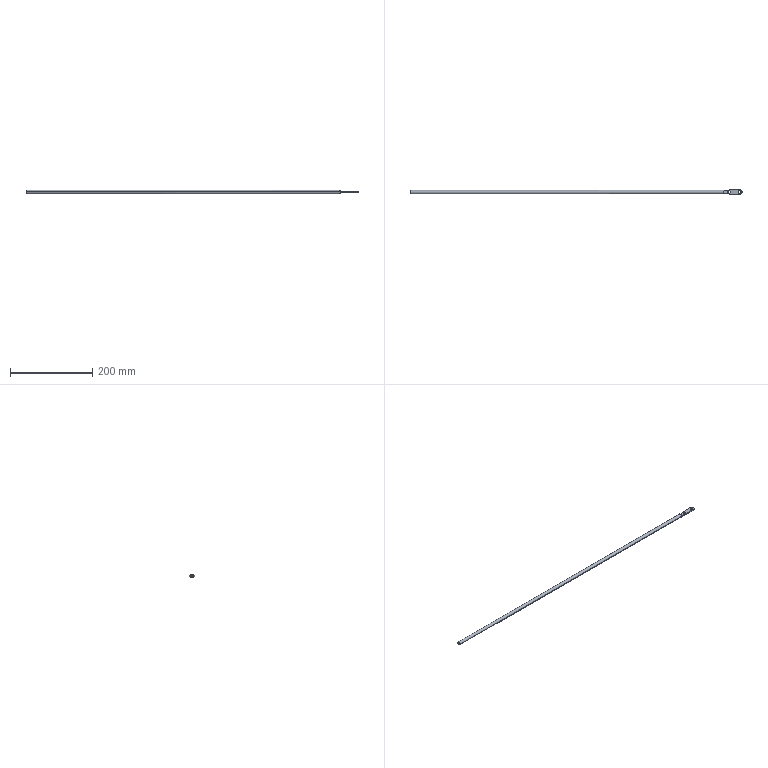Component | SolidWorks | FrontDoorAssembly-1_FrontDoorUpperLockRod-1 | 1 solid | 20 faces | box 806.5 x 13 x 8 mm | volume 39481 mm3 | plane 11 | cylinder 7 | cone 2 | commonest cylinder face diameters 6.5 x4 8 x2 13 x1
build123d program:
from build123d import *

# Parameters (mm, degrees)
SKETCH1_R           = 4
BOSS_EXTRUDE1_DEPTH = 806.5
CUT_EXTRUDE1_DEPTH  = 5
SKETCH3_W           = 42
SKETCH3_H           = 2.024
CUT_EXTRUDE2_DEPTH  = 10
BOSS_EXTRUDE2_DEPTH = 3
CUT_EXTRUDE3_DEPTH  = 3
SKETCH6_R           = 3.25
CUT_EXTRUDE4_DEPTH  = 3
CHAMFER1_SIZE       = 1.5


with BuildPart() as part:
    # Sketch1 → Boss-Extrude1 (new body)
    with BuildSketch(Plane(origin=(0, 0, 0), x_dir=(0, 0, -1), z_dir=(1, 0, 0))):
        Circle(SKETCH1_R)
    extrude(amount=-BOSS_EXTRUDE1_DEPTH)

    # Sketch2 → Cut-Extrude1 (cut, symmetric)
    with BuildSketch(Plane.XY):
        Polygon((-42, 1.5), (-45.678, 4), (-42, 4), (0, 4), (0, 1.5), align=None)
        Polygon((-45.678, -4), (-42, -4), (0, -4), (0, -1.5), (-42, -1.5), align=None)
    extrude(amount=CUT_EXTRUDE1_DEPTH, both=True, mode=Mode.SUBTRACT)

    # Sketch3 → Cut-Extrude2 (cut)
    with BuildSketch(Plane(origin=(0, 1.5, 0), x_dir=(1, 0, 0), z_dir=(0, 1, 0))):
        with Locations((-21, 2.988)):
            Rectangle(SKETCH3_W, SKETCH3_H)
        with Locations((-21, -2.988)):
            Rectangle(SKETCH3_W, SKETCH3_H)
    extrude(amount=-CUT_EXTRUDE2_DEPTH, mode=Mode.SUBTRACT)

    # Sketch4 → Boss-Extrude2 (add)
    with BuildSketch(Plane(origin=(0, 1.5, 0), x_dir=(1, 0, 0), z_dir=(0, 1, 0))):
        with BuildLine():
            Line((-42, -4), (-42, 4))
            Line((-42, 4), (-7.386, 6.439))
            ThreePointArc((-7.386, 6.439), (0, 0), (-7.386, -6.439))
            Line((-7.386, -6.439), (-42, -4))
        make_face()
    extrude(amount=-BOSS_EXTRUDE2_DEPTH)

    # Sketch5 → Cut-Extrude3 (cut)
    with BuildSketch(Plane(origin=(0, 1.5, 0), x_dir=(1, 0, 0), z_dir=(0, 1, 0))):
        with BuildLine():
            Line((-0.8017, 3.127), (2.344, 3.127))
            Line((2.344, 3.127), (2.344, -3.404))
            Line((2.344, -3.404), (-0.9628, -3.404))
            ThreePointArc((-0.9628, -3.404), (-0.001977, -0.1603), (-0.8017, 3.127))
        make_face()
    extrude(amount=-CUT_EXTRUDE3_DEPTH, mode=Mode.SUBTRACT)

    # Sketch6 → Cut-Extrude4 (cut)
    with BuildSketch(Plane(origin=(0, 1.5, 0), x_dir=(1, 0, 0), z_dir=(0, 1, 0))):
        with Locations(Location((-6, 0, 0), (0, 0, 180))):
            Circle(SKETCH6_R)
        with Locations(Location((-31, 0, 0), (0, 0, 180))):
            Circle(SKETCH6_R)
    extrude(amount=-CUT_EXTRUDE4_DEPTH, mode=Mode.SUBTRACT)

    # Chamfer1
    chamfer1_edges = [part.edges().sort_by_distance(p)[0] for p in [
        (-806.5, 0, 4),
    ]]
    chamfer(chamfer1_edges, length=CHAMFER1_SIZE)


solid = part.part

# Placed as in the assembly
solid = solid.moved(Location((-209.186, -273.299, 374.754), (90, 0, 0)))
STEP:
#1=CARTESIAN_POINT('',(-39.988,-10.858,14.754));
#2=VERTEX_POINT('',#1);
#3=CARTESIAN_POINT('',(-39.988,-10.661,14.754));
#4=VERTEX_POINT('',#3);
#5=CARTESIAN_POINT('',(-39.988,-10.76,14.754));
#6=DIRECTION('',(-1.,0.,0.));
#7=DIRECTION('',(0.,1.,0.));
#8=AXIS2_PLACEMENT_3D('',#5,#6,#7);
#9=CIRCLE('',#8,0.09843);
#10=EDGE_CURVE('',#2,#4,#9,.T.);
#11=ORIENTED_EDGE('',*,*,#10,.F.);
#12=CARTESIAN_POINT('',(-39.929,-10.917,14.754));
#13=VERTEX_POINT('',#12);
#14=CARTESIAN_POINT('',(-39.929,-10.917,14.754));
#15=DIRECTION('',(0.7071,-0.7071,-0.));
#16=VECTOR('',#15,39.37);
#17=LINE('',#14,#16);
#18=EDGE_CURVE('',#2,#13,#17,.T.);
#19=ORIENTED_EDGE('',*,*,#18,.T.);
#20=CARTESIAN_POINT('',(-39.929,-10.602,14.754));
#21=VERTEX_POINT('',#20);
#22=CARTESIAN_POINT('',(-39.929,-10.76,14.754));
#23=DIRECTION('',(1.,-0.,-0.));
#24=DIRECTION('',(0.,1.,0.));
#25=AXIS2_PLACEMENT_3D('',#22,#23,#24);
#26=CIRCLE('',#25,0.1575);
#27=EDGE_CURVE('',#21,#13,#26,.T.);
#28=ORIENTED_EDGE('',*,*,#27,.F.);
#29=CARTESIAN_POINT('',(-39.929,-10.602,14.754));
#30=DIRECTION('',(0.7071,0.7071,-0.));
#31=VECTOR('',#30,39.37);
#32=LINE('',#29,#31);
#33=EDGE_CURVE('',#4,#21,#32,.T.);
#34=ORIENTED_EDGE('',*,*,#33,.F.);
#35=EDGE_LOOP('',(#11,#19,#28,#34));
#36=FACE_OUTER_BOUND('',#35,.T.);
#37=CARTESIAN_POINT('',(-39.929,-10.76,14.754));
#38=DIRECTION('',(1.,-0.,-0.));
#39=DIRECTION('',(0.,1.,0.));
#40=AXIS2_PLACEMENT_3D('',#37,#38,#39);
#41=CONICAL_SURFACE('',#40,0.1575,0.7854);
#42=ADVANCED_FACE('',(#36),#41,.T.);
#43=CARTESIAN_POINT('',(-9.328,-10.76,14.695));
#44=VERTEX_POINT('',#43);
#45=CARTESIAN_POINT('',(-9.584,-10.76,14.695));
#46=VERTEX_POINT('',#45);
#47=CARTESIAN_POINT('',(-9.456,-10.76,14.695));
#48=DIRECTION('',(0.,-0.,1.));
#49=DIRECTION('',(-1.,0.,0.));
#50=AXIS2_PLACEMENT_3D('',#47,#48,#49);
#51=CIRCLE('',#50,0.128);
#52=EDGE_CURVE('',#44,#46,#51,.T.);
#53=ORIENTED_EDGE('',*,*,#52,.F.);
#54=CARTESIAN_POINT('',(-9.328,-10.76,14.813));
#55=VERTEX_POINT('',#54);
#56=CARTESIAN_POINT('',(-9.328,-10.76,14.695));
#57=DIRECTION('',(0.,-0.,1.));
#58=VECTOR('',#57,39.37);
#59=LINE('',#56,#58);
#60=EDGE_CURVE('',#44,#55,#59,.T.);
#61=ORIENTED_EDGE('',*,*,#60,.T.);
#62=CARTESIAN_POINT('',(-9.584,-10.76,14.813));
#63=VERTEX_POINT('',#62);
#64=CARTESIAN_POINT('',(-9.456,-10.76,14.813));
#65=DIRECTION('',(0.,-0.,1.));
#66=DIRECTION('',(-1.,0.,0.));
#67=AXIS2_PLACEMENT_3D('',#64,#65,#66);
#68=CIRCLE('',#67,0.128);
#69=EDGE_CURVE('',#55,#63,#68,.T.);
#70=ORIENTED_EDGE('',*,*,#69,.T.);
#71=CARTESIAN_POINT('',(-9.584,-10.76,14.695));
#72=DIRECTION('',(0.,-0.,1.));
#73=VECTOR('',#72,39.37);
#74=LINE('',#71,#73);
#75=EDGE_CURVE('',#46,#63,#74,.T.);
#76=ORIENTED_EDGE('',*,*,#75,.F.);
#77=EDGE_LOOP('',(#53,#61,#70,#76));
#78=FACE_OUTER_BOUND('',#77,.T.);
#79=CARTESIAN_POINT('',(-9.456,-10.76,14.695));
#80=DIRECTION('',(0.,-0.,1.));
#81=DIRECTION('',(-1.,0.,0.));
#82=AXIS2_PLACEMENT_3D('',#79,#80,#81);
#83=CYLINDRICAL_SURFACE('',#82,0.128);
#84=ADVANCED_FACE('',(#78),#83,.F.);
#85=CARTESIAN_POINT('',(-8.344,-10.76,14.695));
#86=VERTEX_POINT('',#85);
#87=CARTESIAN_POINT('',(-8.6,-10.76,14.695));
#88=VERTEX_POINT('',#87);
#89=CARTESIAN_POINT('',(-8.472,-10.76,14.695));
#90=DIRECTION('',(0.,-0.,1.));
#91=DIRECTION('',(-1.,0.,0.));
#92=AXIS2_PLACEMENT_3D('',#89,#90,#91);
#93=CIRCLE('',#92,0.128);
#94=EDGE_CURVE('',#86,#88,#93,.T.);
#95=ORIENTED_EDGE('',*,*,#94,.F.);
#96=CARTESIAN_POINT('',(-8.344,-10.76,14.813));
#97=VERTEX_POINT('',#96);
#98=CARTESIAN_POINT('',(-8.344,-10.76,14.695));
#99=DIRECTION('',(0.,-0.,1.));
#100=VECTOR('',#99,39.37);
#101=LINE('',#98,#100);
#102=EDGE_CURVE('',#86,#97,#101,.T.);
#103=ORIENTED_EDGE('',*,*,#102,.T.);
#104=CARTESIAN_POINT('',(-8.6,-10.76,14.813));
#105=VERTEX_POINT('',#104);
#106=CARTESIAN_POINT('',(-8.472,-10.76,14.813));
#107=DIRECTION('',(0.,-0.,1.));
#108=DIRECTION('',(-1.,0.,0.));
#109=AXIS2_PLACEMENT_3D('',#106,#107,#108);
#110=CIRCLE('',#109,0.128);
#111=EDGE_CURVE('',#97,#105,#110,.T.);
#112=ORIENTED_EDGE('',*,*,#111,.T.);
#113=CARTESIAN_POINT('',(-8.6,-10.76,14.695));
#114=DIRECTION('',(0.,-0.,1.));
#115=VECTOR('',#114,39.37);
#116=LINE('',#113,#115);
#117=EDGE_CURVE('',#88,#105,#116,.T.);
#118=ORIENTED_EDGE('',*,*,#117,.F.);
#119=EDGE_LOOP('',(#95,#103,#112,#118));
#120=FACE_OUTER_BOUND('',#119,.T.);
#121=CARTESIAN_POINT('',(-8.472,-10.76,14.695));
#122=DIRECTION('',(0.,-0.,1.));
#123=DIRECTION('',(-1.,0.,0.));
#124=AXIS2_PLACEMENT_3D('',#121,#122,#123);
#125=CYLINDRICAL_SURFACE('',#124,0.128);
#126=ADVANCED_FACE('',(#120),#125,.F.);
#127=ORIENTED_EDGE('',*,*,#27,.T.);
#128=CARTESIAN_POINT('',(-9.889,-10.917,14.754));
#129=VERTEX_POINT('',#128);
#130=CARTESIAN_POINT('',(-39.988,-10.917,14.754));
#131=DIRECTION('',(1.,-0.,-0.));
#132=VECTOR('',#131,39.37);
#133=LINE('',#130,#132);
#134=EDGE_CURVE('',#13,#129,#133,.T.);
#135=ORIENTED_EDGE('',*,*,#134,.T.);
#136=CARTESIAN_POINT('',(-9.889,-10.906,14.813));
#137=VERTEX_POINT('',#136);
#138=CARTESIAN_POINT('',(-9.889,-10.76,14.754));
#139=DIRECTION('',(1.,-0.,-0.));
#140=DIRECTION('',(0.,0.,-1.));
#141=AXIS2_PLACEMENT_3D('',#138,#139,#140);
#142=CIRCLE('',#141,0.1575);
#143=EDGE_CURVE('',#137,#129,#142,.T.);
#144=ORIENTED_EDGE('',*,*,#143,.F.);
#145=CARTESIAN_POINT('',(-9.889,-10.614,14.813));
#146=VERTEX_POINT('',#145);
#147=CARTESIAN_POINT('',(-9.889,-10.614,14.813));
#148=CARTESIAN_POINT('',(-10.117,-10.676,14.968));
#149=CARTESIAN_POINT('',(-10.117,-10.843,14.968));
#150=CARTESIAN_POINT('',(-9.889,-10.906,14.813));
#151=(BOUNDED_CURVE()B_SPLINE_CURVE(3,(#147,#148,#149,#150),.UNSPECIFIED.,.F.,.F.)B_SPLINE_CURVE_WITH_KNOTS((4,4),(1.955,4.328),.UNSPECIFIED.)CURVE()GEOMETRIC_REPRESENTATION_ITEM()RATIONAL_B_SPLINE_CURVE((1.,0.5833,0.5833,1.))REPRESENTATION_ITEM(''));
#152=EDGE_CURVE('',#146,#137,#151,.T.);
#153=ORIENTED_EDGE('',*,*,#152,.F.);
#154=CARTESIAN_POINT('',(-9.889,-10.602,14.754));
#155=VERTEX_POINT('',#154);
#156=CARTESIAN_POINT('',(-9.889,-10.76,14.754));
#157=DIRECTION('',(1.,-0.,-0.));
#158=DIRECTION('',(0.,0.,-1.));
#159=AXIS2_PLACEMENT_3D('',#156,#157,#158);
#160=CIRCLE('',#159,0.1575);
#161=EDGE_CURVE('',#155,#146,#160,.T.);
#162=ORIENTED_EDGE('',*,*,#161,.F.);
#163=CARTESIAN_POINT('',(-39.988,-10.602,14.754));
#164=DIRECTION('',(1.,-0.,-0.));
#165=VECTOR('',#164,39.37);
#166=LINE('',#163,#165);
#167=EDGE_CURVE('',#21,#155,#166,.T.);
#168=ORIENTED_EDGE('',*,*,#167,.F.);
#169=EDGE_LOOP('',(#127,#135,#144,#153,#162,#168));
#170=FACE_OUTER_BOUND('',#169,.T.);
#171=CARTESIAN_POINT('',(-39.988,-10.76,14.754));
#172=DIRECTION('',(1.,-0.,-0.));
#173=DIRECTION('',(0.,1.,0.));
#174=AXIS2_PLACEMENT_3D('',#171,#172,#173);
#175=CYLINDRICAL_SURFACE('',#174,0.1575);
#176=ADVANCED_FACE('',(#170),#175,.T.);
#177=ORIENTED_EDGE('',*,*,#134,.F.);
#178=CARTESIAN_POINT('',(-39.929,-10.76,14.754));
#179=DIRECTION('',(1.,-0.,-0.));
#180=DIRECTION('',(0.,1.,0.));
#181=AXIS2_PLACEMENT_3D('',#178,#179,#180);
#182=CIRCLE('',#181,0.1575);
#183=EDGE_CURVE('',#13,#21,#182,.T.);
#184=ORIENTED_EDGE('',*,*,#183,.T.);
#185=ORIENTED_EDGE('',*,*,#167,.T.);
#186=CARTESIAN_POINT('',(-9.889,-10.614,14.695));
#187=VERTEX_POINT('',#186);
#188=CARTESIAN_POINT('',(-9.889,-10.76,14.754));
#189=DIRECTION('',(1.,-0.,-0.));
#190=DIRECTION('',(0.,0.,-1.));
#191=AXIS2_PLACEMENT_3D('',#188,#189,#190);
#192=CIRCLE('',#191,0.1575);
#193=EDGE_CURVE('',#187,#155,#192,.T.);
#194=ORIENTED_EDGE('',*,*,#193,.F.);
#195=CARTESIAN_POINT('',(-9.889,-10.906,14.695));
#196=VERTEX_POINT('',#195);
#197=CARTESIAN_POINT('',(-9.889,-10.906,14.695));
#198=CARTESIAN_POINT('',(-10.117,-10.843,14.54));
#199=CARTESIAN_POINT('',(-10.117,-10.676,14.54));
#200=CARTESIAN_POINT('',(-9.889,-10.614,14.695));
#201=(BOUNDED_CURVE()B_SPLINE_CURVE(3,(#197,#198,#199,#200),.UNSPECIFIED.,.F.,.F.)B_SPLINE_CURVE_WITH_KNOTS((4,4),(1.955,4.328),.UNSPECIFIED.)CURVE()GEOMETRIC_REPRESENTATION_ITEM()RATIONAL_B_SPLINE_CURVE((1.,0.5833,0.5833,1.))REPRESENTATION_ITEM(''));
#202=EDGE_CURVE('',#196,#187,#201,.T.);
#203=ORIENTED_EDGE('',*,*,#202,.F.);
#204=CARTESIAN_POINT('',(-9.889,-10.76,14.754));
#205=DIRECTION('',(1.,-0.,-0.));
#206=DIRECTION('',(0.,0.,-1.));
#207=AXIS2_PLACEMENT_3D('',#204,#205,#206);
#208=CIRCLE('',#207,0.1575);
#209=EDGE_CURVE('',#129,#196,#208,.T.);
#210=ORIENTED_EDGE('',*,*,#209,.F.);
#211=EDGE_LOOP('',(#177,#184,#185,#194,#203,#210));
#212=FACE_OUTER_BOUND('',#211,.T.);
#213=CARTESIAN_POINT('',(-39.988,-10.76,14.754));
#214=DIRECTION('',(1.,-0.,-0.));
#215=DIRECTION('',(0.,1.,0.));
#216=AXIS2_PLACEMENT_3D('',#213,#214,#215);
#217=CYLINDRICAL_SURFACE('',#216,0.1575);
#218=ADVANCED_FACE('',(#212),#217,.T.);
#219=CARTESIAN_POINT('',(-39.988,-10.76,14.754));
#220=DIRECTION('',(-1.,0.,0.));
#221=DIRECTION('',(0.,1.,0.));
#222=AXIS2_PLACEMENT_3D('',#219,#220,#221);
#223=CIRCLE('',#222,0.09843);
#224=EDGE_CURVE('',#4,#2,#223,.T.);
#225=ORIENTED_EDGE('',*,*,#224,.T.);
#226=ORIENTED_EDGE('',*,*,#10,.T.);
#227=EDGE_LOOP('',(#225,#226));
#228=FACE_OUTER_BOUND('',#227,.T.);
#229=CARTESIAN_POINT('',(-39.988,-10.76,14.754));
#230=DIRECTION('',(1.,-0.,-0.));
#231=DIRECTION('',(0.,1.,0.));
#232=AXIS2_PLACEMENT_3D('',#229,#230,#231);
#233=PLANE('',#232);
#234=ADVANCED_FACE('',(#228),#233,.F.);
#235=CARTESIAN_POINT('',(-9.456,-10.76,14.813));
#236=DIRECTION('',(0.,-0.,1.));
#237=DIRECTION('',(-1.,0.,0.));
#238=AXIS2_PLACEMENT_3D('',#235,#236,#237);
#239=CIRCLE('',#238,0.128);
#240=EDGE_CURVE('',#63,#55,#239,.T.);
#241=ORIENTED_EDGE('',*,*,#240,.F.);
#242=ORIENTED_EDGE('',*,*,#69,.F.);
#243=EDGE_LOOP('',(#241,#242));
#244=FACE_BOUND('',#243,.T.);
#245=CARTESIAN_POINT('',(-8.472,-10.76,14.813));
#246=DIRECTION('',(0.,-0.,1.));
#247=DIRECTION('',(-1.,0.,0.));
#248=AXIS2_PLACEMENT_3D('',#245,#246,#247);
#249=CIRCLE('',#248,0.128);
#250=EDGE_CURVE('',#105,#97,#249,.T.);
#251=ORIENTED_EDGE('',*,*,#250,.F.);
#252=ORIENTED_EDGE('',*,*,#111,.F.);
#253=EDGE_LOOP('',(#251,#252));
#254=FACE_BOUND('',#253,.T.);
#255=CARTESIAN_POINT('',(-9.889,-10.917,14.813));
#256=VERTEX_POINT('',#255);
#257=CARTESIAN_POINT('',(-8.526,-11.013,14.813));
#258=VERTEX_POINT('',#257);
#259=CARTESIAN_POINT('',(-9.889,-10.917,14.813));
#260=DIRECTION('',(0.9975,-0.0703,-0.));
#261=VECTOR('',#260,39.37);
#262=LINE('',#259,#261);
#263=EDGE_CURVE('',#256,#258,#262,.T.);
#264=ORIENTED_EDGE('',*,*,#263,.T.);
#265=CARTESIAN_POINT('',(-8.526,-10.506,14.813));
#266=VERTEX_POINT('',#265);
#267=CARTESIAN_POINT('',(-8.492,-10.76,14.813));
#268=DIRECTION('',(0.,-0.,1.));
#269=DIRECTION('',(-1.,0.,0.));
#270=AXIS2_PLACEMENT_3D('',#267,#268,#269);
#271=CIRCLE('',#270,0.2559);
#272=EDGE_CURVE('',#258,#266,#271,.T.);
#273=ORIENTED_EDGE('',*,*,#272,.T.);
#274=CARTESIAN_POINT('',(-9.889,-10.602,14.813));
#275=VERTEX_POINT('',#274);
#276=CARTESIAN_POINT('',(-9.889,-10.602,14.813));
#277=DIRECTION('',(-0.9975,-0.0703,0.));
#278=VECTOR('',#277,39.37);
#279=LINE('',#276,#278);
#280=EDGE_CURVE('',#266,#275,#279,.T.);
#281=ORIENTED_EDGE('',*,*,#280,.T.);
#282=CARTESIAN_POINT('',(-9.889,-10.917,14.813));
#283=DIRECTION('',(-0.,-1.,-0.));
#284=VECTOR('',#283,39.37);
#285=LINE('',#282,#284);
#286=EDGE_CURVE('',#275,#146,#285,.T.);
#287=ORIENTED_EDGE('',*,*,#286,.T.);
#288=CARTESIAN_POINT('',(-9.889,-10.563,14.813));
#289=DIRECTION('',(-0.,-1.,-0.));
#290=VECTOR('',#289,39.37);
#291=LINE('',#288,#290);
#292=EDGE_CURVE('',#146,#137,#291,.T.);
#293=ORIENTED_EDGE('',*,*,#292,.T.);
#294=CARTESIAN_POINT('',(-9.889,-10.917,14.813));
#295=DIRECTION('',(-0.,-1.,-0.));
#296=VECTOR('',#295,39.37);
#297=LINE('',#294,#296);
#298=EDGE_CURVE('',#137,#256,#297,.T.);
#299=ORIENTED_EDGE('',*,*,#298,.T.);
#300=EDGE_LOOP('',(#264,#273,#281,#287,#293,#299));
#301=FACE_OUTER_BOUND('',#300,.T.);
#302=CARTESIAN_POINT('',(-8.236,-10.563,14.813));
#303=DIRECTION('',(-0.,0.,-1.));
#304=DIRECTION('',(1.,-0.,-0.));
#305=AXIS2_PLACEMENT_3D('',#302,#303,#304);
#306=PLANE('',#305);
#307=ADVANCED_FACE('',(#244,#254,#301),#306,.F.);
#308=ORIENTED_EDGE('',*,*,#292,.F.);
#309=ORIENTED_EDGE('',*,*,#152,.T.);
#310=EDGE_LOOP('',(#308,#309));
#311=FACE_OUTER_BOUND('',#310,.T.);
#312=CARTESIAN_POINT('',(-9.889,-10.563,14.813));
#313=DIRECTION('',(-0.5621,0.,-0.8271));
#314=DIRECTION('',(0.8271,-0.,-0.5621));
#315=AXIS2_PLACEMENT_3D('',#312,#313,#314);
#316=PLANE('',#315);
#317=ADVANCED_FACE('',(#311),#316,.F.);
#318=CARTESIAN_POINT('',(-9.889,-10.563,14.695));
#319=DIRECTION('',(-0.,-1.,-0.));
#320=VECTOR('',#319,39.37);
#321=LINE('',#318,#320);
#322=EDGE_CURVE('',#187,#196,#321,.T.);
#323=ORIENTED_EDGE('',*,*,#322,.T.);
#324=ORIENTED_EDGE('',*,*,#202,.T.);
#325=EDGE_LOOP('',(#323,#324));
#326=FACE_OUTER_BOUND('',#325,.T.);
#327=CARTESIAN_POINT('',(-9.889,-10.563,14.695));
#328=DIRECTION('',(-0.5621,0.,0.8271));
#329=DIRECTION('',(-0.8271,0.,-0.5621));
#330=AXIS2_PLACEMENT_3D('',#327,#328,#329);
#331=PLANE('',#330);
#332=ADVANCED_FACE('',(#326),#331,.F.);
#333=CARTESIAN_POINT('',(-9.456,-10.76,14.695));
#334=DIRECTION('',(0.,-0.,1.));
#335=DIRECTION('',(-1.,0.,0.));
#336=AXIS2_PLACEMENT_3D('',#333,#334,#335);
#337=CIRCLE('',#336,0.128);
#338=EDGE_CURVE('',#46,#44,#337,.T.);
#339=ORIENTED_EDGE('',*,*,#338,.T.);
#340=ORIENTED_EDGE('',*,*,#52,.T.);
#341=EDGE_LOOP('',(#339,#340));
#342=FACE_BOUND('',#341,.T.);
#343=CARTESIAN_POINT('',(-8.472,-10.76,14.695));
#344=DIRECTION('',(0.,-0.,1.));
#345=DIRECTION('',(-1.,0.,0.));
#346=AXIS2_PLACEMENT_3D('',#343,#344,#345);
#347=CIRCLE('',#346,0.128);
#348=EDGE_CURVE('',#88,#86,#347,.T.);
#349=ORIENTED_EDGE('',*,*,#348,.T.);
#350=ORIENTED_EDGE('',*,*,#94,.T.);
#351=EDGE_LOOP('',(#349,#350));
#352=FACE_BOUND('',#351,.T.);
#353=CARTESIAN_POINT('',(-8.526,-11.013,14.695));
#354=VERTEX_POINT('',#353);
#355=CARTESIAN_POINT('',(-8.526,-10.506,14.695));
#356=VERTEX_POINT('',#355);
#357=CARTESIAN_POINT('',(-8.492,-10.76,14.695));
#358=DIRECTION('',(0.,-0.,1.));
#359=DIRECTION('',(-1.,0.,0.));
#360=AXIS2_PLACEMENT_3D('',#357,#358,#359);
#361=CIRCLE('',#360,0.2559);
#362=EDGE_CURVE('',#354,#356,#361,.T.);
#363=ORIENTED_EDGE('',*,*,#362,.F.);
#364=CARTESIAN_POINT('',(-9.889,-10.917,14.695));
#365=VERTEX_POINT('',#364);
#366=CARTESIAN_POINT('',(-9.889,-10.917,14.695));
#367=DIRECTION('',(0.9975,-0.0703,-0.));
#368=VECTOR('',#367,39.37);
#369=LINE('',#366,#368);
#370=EDGE_CURVE('',#365,#354,#369,.T.);
#371=ORIENTED_EDGE('',*,*,#370,.F.);
#372=CARTESIAN_POINT('',(-9.889,-10.917,14.695));
#373=DIRECTION('',(-0.,-1.,-0.));
#374=VECTOR('',#373,39.37);
#375=LINE('',#372,#374);
#376=EDGE_CURVE('',#196,#365,#375,.T.);
#377=ORIENTED_EDGE('',*,*,#376,.F.);
#378=ORIENTED_EDGE('',*,*,#322,.F.);
#379=CARTESIAN_POINT('',(-9.889,-10.602,14.695));
#380=VERTEX_POINT('',#379);
#381=CARTESIAN_POINT('',(-9.889,-10.917,14.695));
#382=DIRECTION('',(-0.,-1.,-0.));
#383=VECTOR('',#382,39.37);
#384=LINE('',#381,#383);
#385=EDGE_CURVE('',#380,#187,#384,.T.);
#386=ORIENTED_EDGE('',*,*,#385,.F.);
#387=CARTESIAN_POINT('',(-9.889,-10.602,14.695));
#388=DIRECTION('',(-0.9975,-0.0703,0.));
#389=VECTOR('',#388,39.37);
#390=LINE('',#387,#389);
#391=EDGE_CURVE('',#356,#380,#390,.T.);
#392=ORIENTED_EDGE('',*,*,#391,.F.);
#393=EDGE_LOOP('',(#363,#371,#377,#378,#386,#392));
#394=FACE_OUTER_BOUND('',#393,.T.);
#395=CARTESIAN_POINT('',(-8.236,-10.563,14.695));
#396=DIRECTION('',(0.,-0.,1.));
#397=DIRECTION('',(-1.,0.,0.));
#398=AXIS2_PLACEMENT_3D('',#395,#396,#397);
#399=PLANE('',#398);
#400=ADVANCED_FACE('',(#342,#352,#394),#399,.F.);
#401=ORIENTED_EDGE('',*,*,#263,.F.);
#402=CARTESIAN_POINT('',(-9.889,-10.917,14.695));
#403=DIRECTION('',(0.,-0.,1.));
#404=VECTOR('',#403,39.37);
#405=LINE('',#402,#404);
#406=EDGE_CURVE('',#129,#256,#405,.T.);
#407=ORIENTED_EDGE('',*,*,#406,.F.);
#408=CARTESIAN_POINT('',(-9.889,-10.917,14.695));
#409=DIRECTION('',(0.,-0.,1.));
#410=VECTOR('',#409,39.37);
#411=LINE('',#408,#410);
#412=EDGE_CURVE('',#365,#129,#411,.T.);
#413=ORIENTED_EDGE('',*,*,#412,.F.);
#414=ORIENTED_EDGE('',*,*,#370,.T.);
#415=CARTESIAN_POINT('',(-8.526,-11.013,14.695));
#416=DIRECTION('',(0.,-0.,1.));
#417=VECTOR('',#416,39.37);
#418=LINE('',#415,#417);
#419=EDGE_CURVE('',#354,#258,#418,.T.);
#420=ORIENTED_EDGE('',*,*,#419,.T.);
#421=EDGE_LOOP('',(#401,#407,#413,#414,#420));
#422=FACE_OUTER_BOUND('',#421,.T.);
#423=CARTESIAN_POINT('',(-9.889,-10.917,14.695));
#424=DIRECTION('',(-0.0703,-0.9975,-0.));
#425=DIRECTION('',(0.9975,-0.0703,-0.));
#426=AXIS2_PLACEMENT_3D('',#423,#424,#425);
#427=PLANE('',#426);
#428=ADVANCED_FACE('',(#422),#427,.T.);
#429=ORIENTED_EDGE('',*,*,#412,.T.);
#430=ORIENTED_EDGE('',*,*,#209,.T.);
#431=ORIENTED_EDGE('',*,*,#376,.T.);
#432=EDGE_LOOP('',(#429,#430,#431));
#433=FACE_OUTER_BOUND('',#432,.T.);
#434=CARTESIAN_POINT('',(-9.889,-10.917,14.695));
#435=DIRECTION('',(-1.,0.,0.));
#436=DIRECTION('',(-0.,0.,-1.));
#437=AXIS2_PLACEMENT_3D('',#434,#435,#436);
#438=PLANE('',#437);
#439=ADVANCED_FACE('',(#433),#438,.T.);
#440=ORIENTED_EDGE('',*,*,#298,.F.);
#441=ORIENTED_EDGE('',*,*,#143,.T.);
#442=ORIENTED_EDGE('',*,*,#406,.T.);
#443=EDGE_LOOP('',(#440,#441,#442));
#444=FACE_OUTER_BOUND('',#443,.T.);
#445=CARTESIAN_POINT('',(-9.889,-10.917,14.695));
#446=DIRECTION('',(-1.,0.,0.));
#447=DIRECTION('',(-0.,0.,-1.));
#448=AXIS2_PLACEMENT_3D('',#445,#446,#447);
#449=PLANE('',#448);
#450=ADVANCED_FACE('',(#444),#449,.T.);
#451=ORIENTED_EDGE('',*,*,#385,.T.);
#452=ORIENTED_EDGE('',*,*,#193,.T.);
#453=CARTESIAN_POINT('',(-9.889,-10.602,14.695));
#454=DIRECTION('',(0.,-0.,1.));
#455=VECTOR('',#454,39.37);
#456=LINE('',#453,#455);
#457=EDGE_CURVE('',#380,#155,#456,.T.);
#458=ORIENTED_EDGE('',*,*,#457,.F.);
#459=EDGE_LOOP('',(#451,#452,#458));
#460=FACE_OUTER_BOUND('',#459,.T.);
#461=CARTESIAN_POINT('',(-9.889,-10.917,14.695));
#462=DIRECTION('',(-1.,0.,0.));
#463=DIRECTION('',(-0.,0.,-1.));
#464=AXIS2_PLACEMENT_3D('',#461,#462,#463);
#465=PLANE('',#464);
#466=ADVANCED_FACE('',(#460),#465,.T.);
#467=CARTESIAN_POINT('',(-9.889,-10.602,14.695));
#468=DIRECTION('',(0.,-0.,1.));
#469=VECTOR('',#468,39.37);
#470=LINE('',#467,#469);
#471=EDGE_CURVE('',#155,#275,#470,.T.);
#472=ORIENTED_EDGE('',*,*,#471,.F.);
#473=ORIENTED_EDGE('',*,*,#161,.T.);
#474=ORIENTED_EDGE('',*,*,#286,.F.);
#475=EDGE_LOOP('',(#472,#473,#474));
#476=FACE_OUTER_BOUND('',#475,.T.);
#477=CARTESIAN_POINT('',(-9.889,-10.917,14.695));
#478=DIRECTION('',(-1.,0.,0.));
#479=DIRECTION('',(-0.,0.,-1.));
#480=AXIS2_PLACEMENT_3D('',#477,#478,#479);
#481=PLANE('',#480);
#482=ADVANCED_FACE('',(#476),#481,.T.);
#483=CARTESIAN_POINT('',(-8.526,-10.506,14.695));
#484=DIRECTION('',(0.,-0.,1.));
#485=VECTOR('',#484,39.37);
#486=LINE('',#483,#485);
#487=EDGE_CURVE('',#356,#266,#486,.T.);
#488=ORIENTED_EDGE('',*,*,#487,.T.);
#489=ORIENTED_EDGE('',*,*,#272,.F.);
#490=ORIENTED_EDGE('',*,*,#419,.F.);
#491=ORIENTED_EDGE('',*,*,#362,.T.);
#492=EDGE_LOOP('',(#488,#489,#490,#491));
#493=FACE_OUTER_BOUND('',#492,.T.);
#494=CARTESIAN_POINT('',(-8.492,-10.76,14.695));
#495=DIRECTION('',(0.,-0.,1.));
#496=DIRECTION('',(-1.,0.,0.));
#497=AXIS2_PLACEMENT_3D('',#494,#495,#496);
#498=CYLINDRICAL_SURFACE('',#497,0.2559);
#499=ADVANCED_FACE('',(#493),#498,.T.);
#500=ORIENTED_EDGE('',*,*,#280,.F.);
#501=ORIENTED_EDGE('',*,*,#487,.F.);
#502=ORIENTED_EDGE('',*,*,#391,.T.);
#503=ORIENTED_EDGE('',*,*,#457,.T.);
#504=ORIENTED_EDGE('',*,*,#471,.T.);
#505=EDGE_LOOP('',(#500,#501,#502,#503,#504));
#506=FACE_OUTER_BOUND('',#505,.T.);
#507=CARTESIAN_POINT('',(-9.889,-10.602,14.695));
#508=DIRECTION('',(-0.0703,0.9975,0.));
#509=DIRECTION('',(-0.9975,-0.0703,0.));
#510=AXIS2_PLACEMENT_3D('',#507,#508,#509);
#511=PLANE('',#510);
#512=ADVANCED_FACE('',(#506),#511,.T.);
#513=ORIENTED_EDGE('',*,*,#102,.F.);
#514=ORIENTED_EDGE('',*,*,#348,.F.);
#515=ORIENTED_EDGE('',*,*,#117,.T.);
#516=ORIENTED_EDGE('',*,*,#250,.T.);
#517=EDGE_LOOP('',(#513,#514,#515,#516));
#518=FACE_OUTER_BOUND('',#517,.T.);
#519=CARTESIAN_POINT('',(-8.472,-10.76,14.695));
#520=DIRECTION('',(0.,-0.,1.));
#521=DIRECTION('',(-1.,0.,0.));
#522=AXIS2_PLACEMENT_3D('',#519,#520,#521);
#523=CYLINDRICAL_SURFACE('',#522,0.128);
#524=ADVANCED_FACE('',(#518),#523,.F.);
#525=ORIENTED_EDGE('',*,*,#60,.F.);
#526=ORIENTED_EDGE('',*,*,#338,.F.);
#527=ORIENTED_EDGE('',*,*,#75,.T.);
#528=ORIENTED_EDGE('',*,*,#240,.T.);
#529=EDGE_LOOP('',(#525,#526,#527,#528));
#530=FACE_OUTER_BOUND('',#529,.T.);
#531=CARTESIAN_POINT('',(-9.456,-10.76,14.695));
#532=DIRECTION('',(0.,-0.,1.));
#533=DIRECTION('',(-1.,0.,0.));
#534=AXIS2_PLACEMENT_3D('',#531,#532,#533);
#535=CYLINDRICAL_SURFACE('',#534,0.128);
#536=ADVANCED_FACE('',(#530),#535,.F.);
#537=ORIENTED_EDGE('',*,*,#18,.F.);
#538=ORIENTED_EDGE('',*,*,#224,.F.);
#539=ORIENTED_EDGE('',*,*,#33,.T.);
#540=ORIENTED_EDGE('',*,*,#183,.F.);
#541=EDGE_LOOP('',(#537,#538,#539,#540));
#542=FACE_OUTER_BOUND('',#541,.T.);
#543=CARTESIAN_POINT('',(-39.929,-10.76,14.754));
#544=DIRECTION('',(1.,-0.,-0.));
#545=DIRECTION('',(0.,1.,0.));
#546=AXIS2_PLACEMENT_3D('',#543,#544,#545);
#547=CONICAL_SURFACE('',#546,0.1575,0.7854);
#548=ADVANCED_FACE('',(#542),#547,.T.);
#549=CLOSED_SHELL('',(#42,#84,#126,#176,#218,#234,#307,#317,#332,#400,#428,#439,#450,#466,#482,#499,#512,#524,#536,#548));
#550=MANIFOLD_SOLID_BREP('',#549);
#551=CARTESIAN_POINT('',(0.,0.,0.));
#552=DIRECTION('',(0.,0.,1.));
#553=DIRECTION('',(1.,0.,0.));
#554=AXIS2_PLACEMENT_3D('',#551,#552,#553);
#555=(LENGTH_UNIT()NAMED_UNIT(*)SI_UNIT($,.METRE.));
#556=LENGTH_MEASURE_WITH_UNIT(LENGTH_MEASURE(0.0254),#555);
#557=DIMENSIONAL_EXPONENTS(1.,0.,0.,0.,0.,0.,0.);
#558=(CONVERSION_BASED_UNIT('',#556)LENGTH_UNIT()NAMED_UNIT(#557));
#559=UNCERTAINTY_MEASURE_WITH_UNIT(LENGTH_MEASURE(0.00001),#558,'','');
#560=(NAMED_UNIT(*)PLANE_ANGLE_UNIT()SI_UNIT($,.RADIAN.));
#561=(NAMED_UNIT(*)SI_UNIT($,.STERADIAN.)SOLID_ANGLE_UNIT());
#562=(GEOMETRIC_REPRESENTATION_CONTEXT(3)GLOBAL_UNCERTAINTY_ASSIGNED_CONTEXT((#559))GLOBAL_UNIT_ASSIGNED_CONTEXT((#558,#560,#561))REPRESENTATION_CONTEXT('',''));
#563=ADVANCED_BREP_SHAPE_REPRESENTATION('',(#550,#554),#562);
#564=COLOUR_RGB('',0.7922,0.8196,0.9333);
#565=FILL_AREA_STYLE_COLOUR('',#564);
#566=FILL_AREA_STYLE('',(#565));
#567=SURFACE_STYLE_FILL_AREA(#566);
#568=SURFACE_SIDE_STYLE('',(#567));
#569=SURFACE_STYLE_USAGE(.BOTH.,#568);
#570=PRESENTATION_STYLE_ASSIGNMENT((#569));
#571=STYLED_ITEM('',(#570),#550);
#572=PRESENTATION_LAYER_ASSIGNMENT('','',(#571));
#573=(LENGTH_UNIT()NAMED_UNIT(*)SI_UNIT($,.METRE.));
#574=LENGTH_MEASURE_WITH_UNIT(LENGTH_MEASURE(0.0254),#573);
#575=DIMENSIONAL_EXPONENTS(1.,0.,0.,0.,0.,0.,0.);
#576=(CONVERSION_BASED_UNIT('',#574)LENGTH_UNIT()NAMED_UNIT(#575));
#577=UNCERTAINTY_MEASURE_WITH_UNIT(LENGTH_MEASURE(0.00001),#576,'','');
#578=(NAMED_UNIT(*)PLANE_ANGLE_UNIT()SI_UNIT($,.RADIAN.));
#579=(NAMED_UNIT(*)SI_UNIT($,.STERADIAN.)SOLID_ANGLE_UNIT());
#580=(GEOMETRIC_REPRESENTATION_CONTEXT(3)GLOBAL_UNCERTAINTY_ASSIGNED_CONTEXT((#577))GLOBAL_UNIT_ASSIGNED_CONTEXT((#576,#578,#579))REPRESENTATION_CONTEXT('',''));
#581=MECHANICAL_DESIGN_GEOMETRIC_PRESENTATION_REPRESENTATION('',(#571),#580);